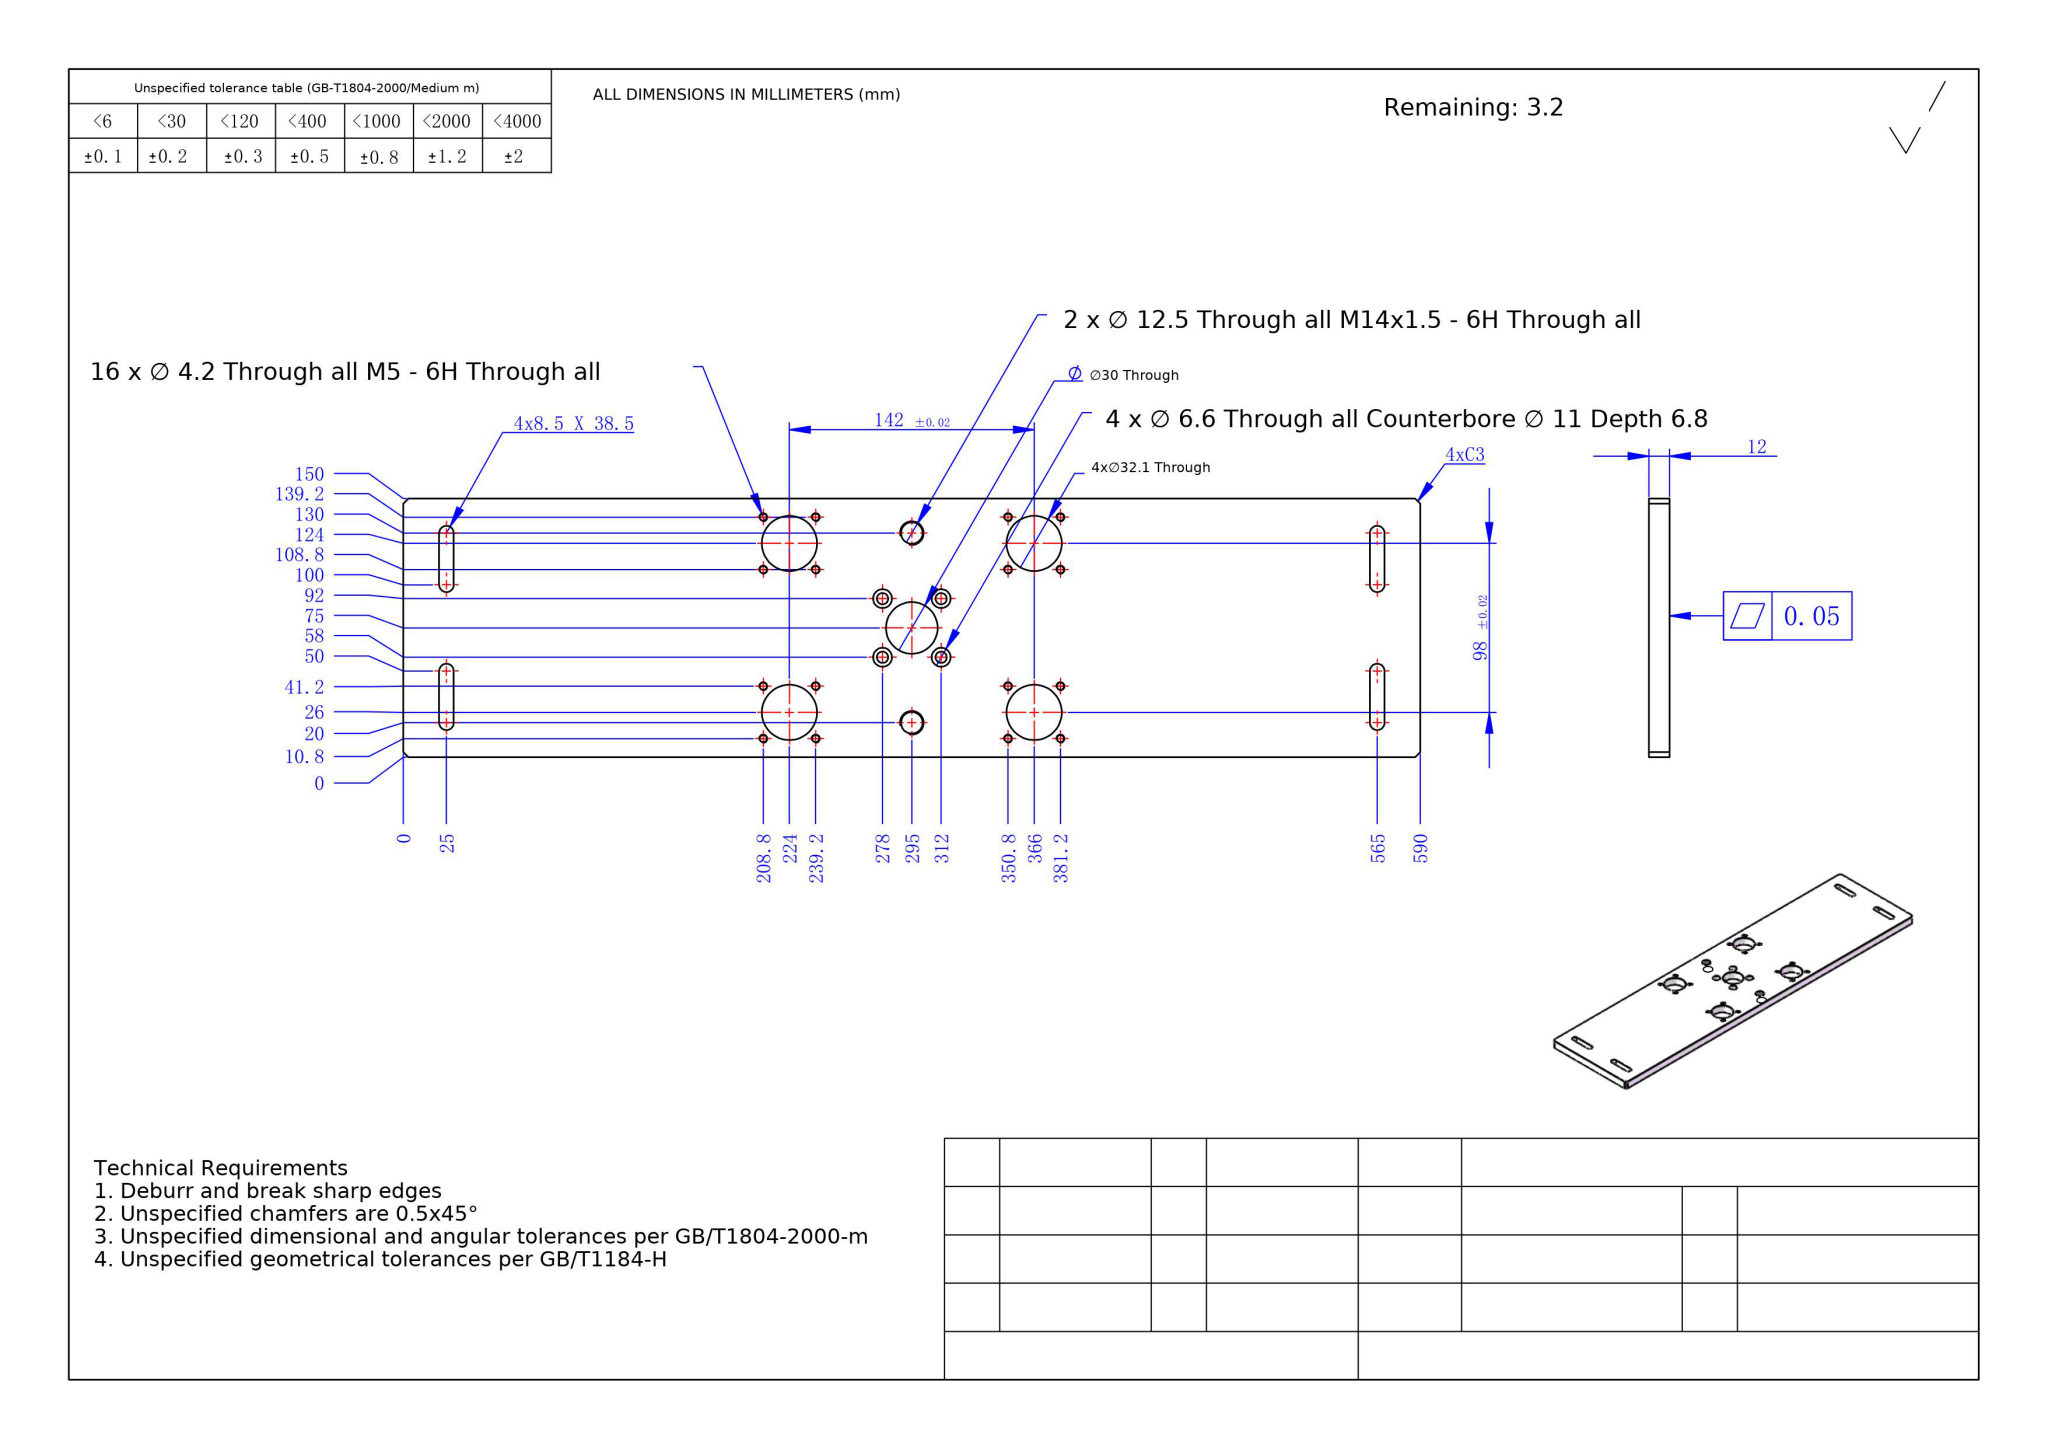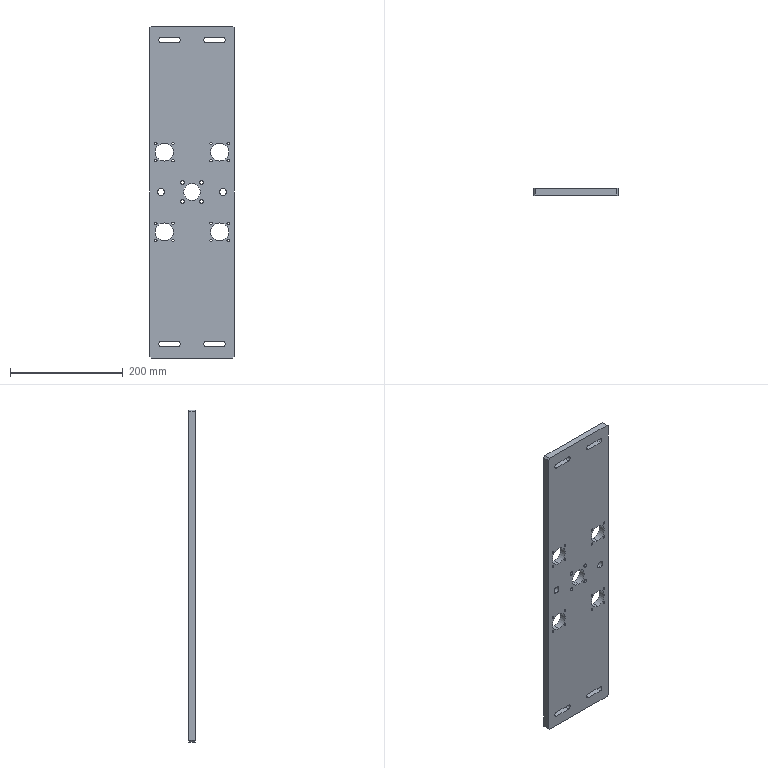Part | NX | mm | 1 solid | 92 faces | box 150 x 12 x 590 mm | volume 990591 mm3 | cylinder 70 | plane 22 | commonest cylinder face diameters 4.2 x32 11 x8 6.6 x8 32.1 x8 8.5 x8 12.5 x4 30 x2